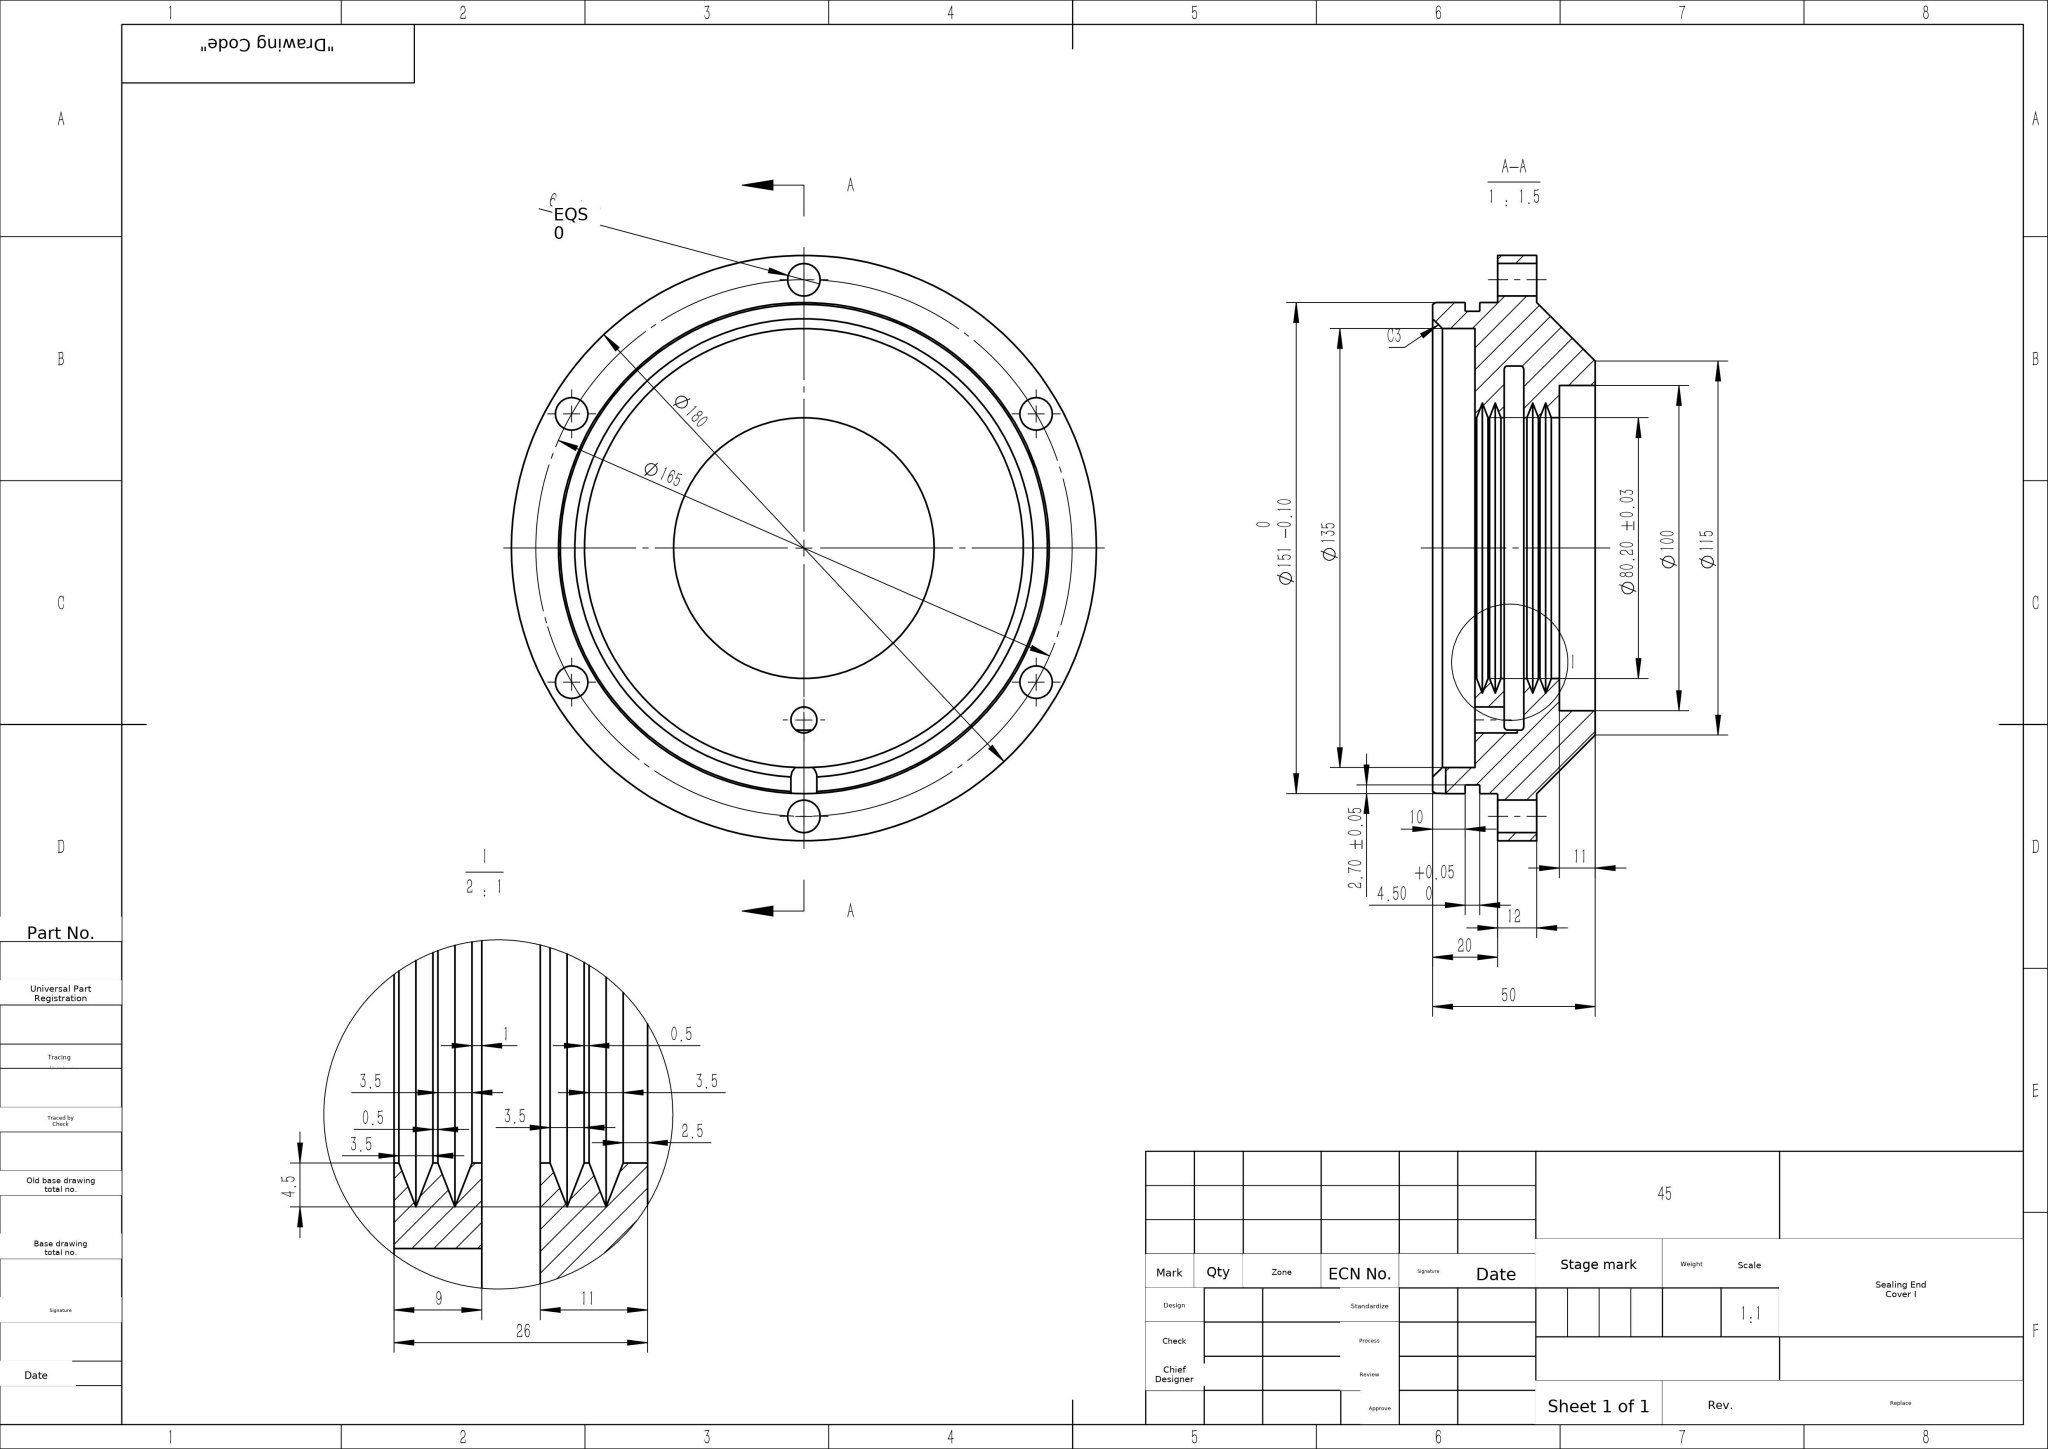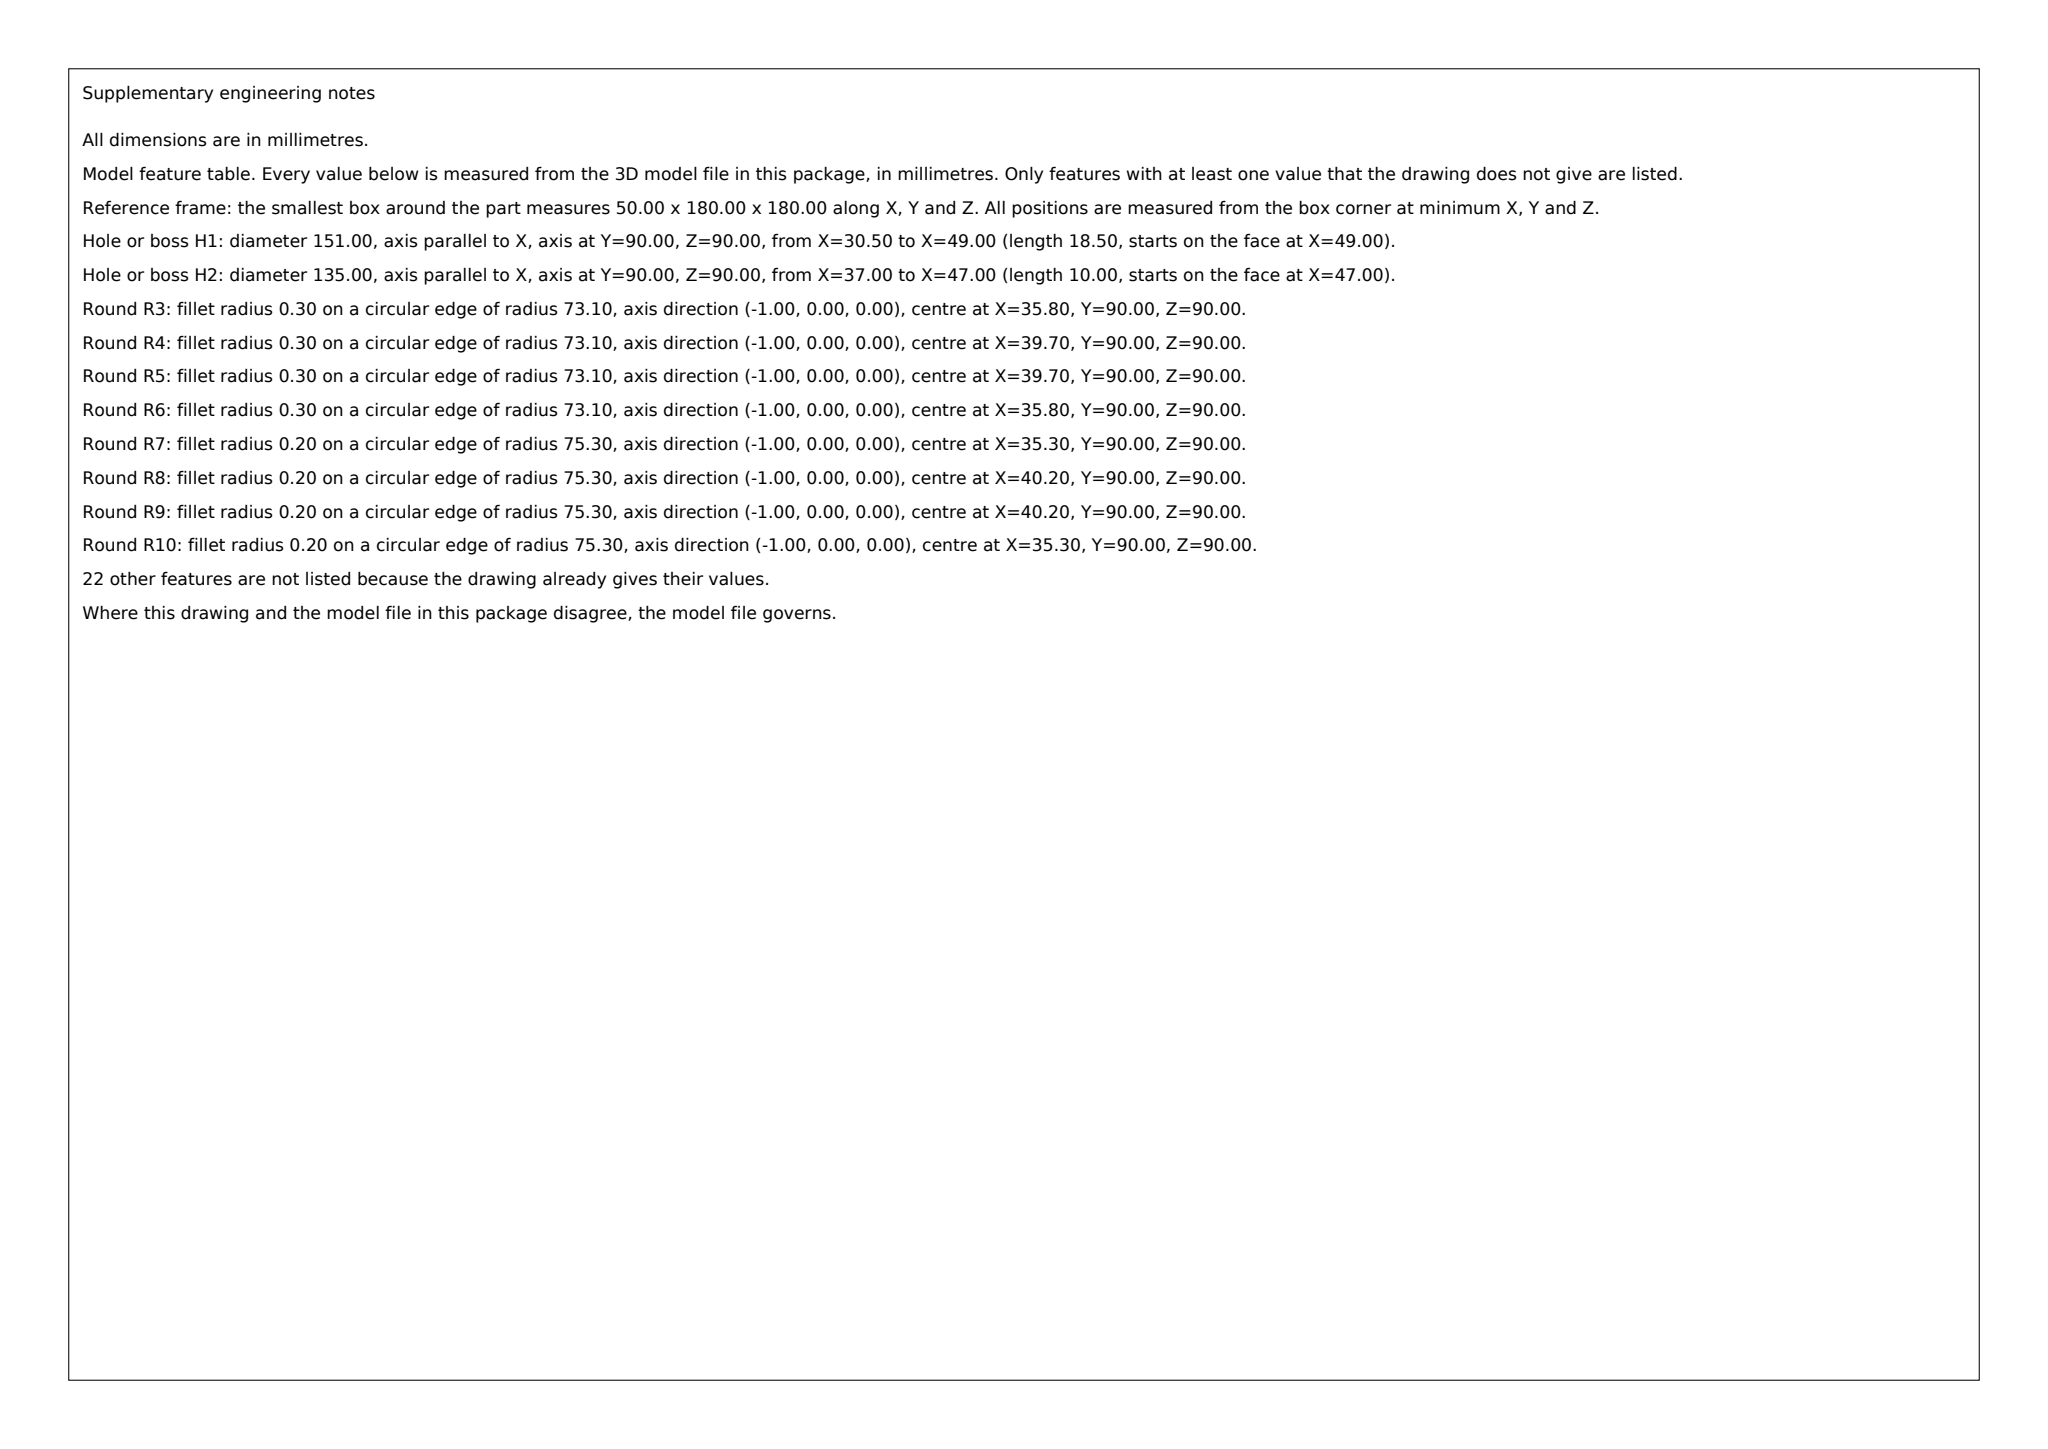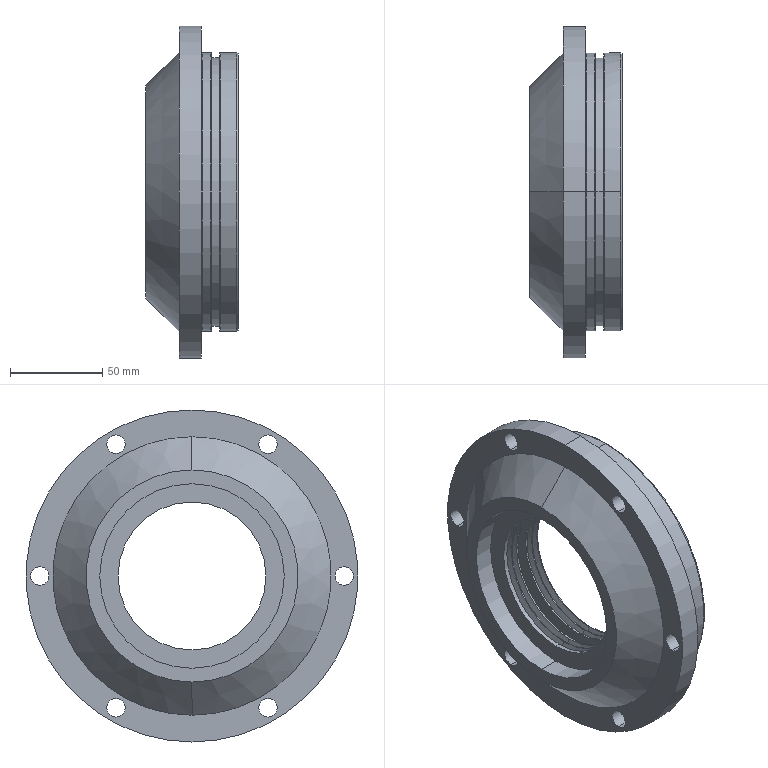Part | SolidWorks | mm | 1 solid | 91 faces | box 50 x 180 x 180 mm | volume 460431 mm3 | cylinder 41 | cone 24 | torus 15 | plane 11 | commonest cylinder face diameters 10 x12 80.2 x12 151 x4 8 x3 100 x2 180 x2 145.6 x2 112 x2
build123d program:
from build123d import *

# Parameters (mm, degrees)
SKETCH2_R          = 5
CUT_EXTRUDE1_DEPTH = 131.767
CHAMFER1_SIZE      = 3
SKETCH3_R          = 4
CUT_EXTRUDE2_DEPTH = 13
SKETCH4_R          = 4
CUT_EXTRUDE3_DEPTH = 134.12


with BuildPart() as part:
    # Sketch1 → Revolve1 (revolve)
    with BuildSketch(Plane.XY, mode=Mode.PRIVATE) as revolve1_sk:
        with BuildLine():
            Line((7, 90), (19, 90))
            Line((19, 90), (19, 76))
            ThreePointArc((19, 76), (19.146, 75.646), (19.5, 75.5))
            Line((19.5, 75.5), (24.3, 75.5))
            ThreePointArc((24.3, 75.5), (24.441, 75.441), (24.5, 75.3))
            Line((24.5, 75.3), (24.5, 73.1))
            ThreePointArc((24.5, 73.1), (24.588, 72.888), (24.8, 72.8))
            Line((24.8, 72.8), (28.7, 72.8))
            ThreePointArc((28.7, 72.8), (28.912, 72.888), (29, 73.1))
            Line((29, 73.1), (29, 75.3))
            ThreePointArc((29, 75.3), (29.059, 75.441), (29.2, 75.5))
            Line((29.2, 75.5), (38, 75.5))
            Line((38, 75.5), (39, 74.923))
            Line((39, 74.923), (39, 67.5))
            Line((39, 67.5), (26, 67.5))
            Line((26, 67.5), (26, 40.1))
            Line((26, 40.1), (25.5, 40.1))
            Line((25.5, 40.1), (23.75, 44.6))
            Line((23.75, 44.6), (22, 40.1))
            Line((22, 40.1), (21.5, 40.1))
            Line((21.5, 40.1), (19.75, 44.6))
            Line((19.75, 44.6), (18, 40.1))
            Line((18, 40.1), (17, 40.1))
            Line((17, 40.1), (17, 55))
            ThreePointArc((17, 55), (16.707, 55.707), (16, 56))
            Line((16, 56), (12, 56))
            ThreePointArc((12, 56), (11.293, 55.707), (11, 55))
            Line((11, 55), (11, 40.1))
            Line((11, 40.1), (10, 40.1))
            Line((10, 40.1), (8.25, 44.6))
            Line((8.25, 44.6), (6.5, 40.1))
            Line((6.5, 40.1), (6, 40.1))
            Line((6, 40.1), (4.25, 44.6))
            Line((4.25, 44.6), (2.5, 40.1))
            Line((2.5, 40.1), (0, 40.1))
            Line((0, 40.1), (0, 50))
            Line((0, 50), (-11, 50))
            Line((-11, 50), (-11, 57.5))
            Line((-11, 57.5), (7, 75.5))
            Line((7, 75.5), (7, 90))
        make_face()
    revolve(revolve1_sk.sketch.rotate(Axis((0, 0, 0), (1, 0, 0)), 90), axis=Axis((0, 0, 0), (1, 0, 0)))

    # Sketch2 → Cut-Extrude1 (cut, through all)
    with BuildSketch(Plane(origin=(19, 0, 0), x_dir=(0, 0, -1), z_dir=(1, 0, 0))):
        with Locations((0, 82.5)):
            Circle(SKETCH2_R)
        with Locations((71.447, 41.25)):
            Circle(SKETCH2_R)
        with Locations((71.447, -41.25)):
            Circle(SKETCH2_R)
        with Locations((0, -82.5)):
            Circle(SKETCH2_R)
        with Locations((-71.447, -41.25)):
            Circle(SKETCH2_R)
        with Locations((-71.447, 41.25)):
            Circle(SKETCH2_R)
    extrude(amount=-CUT_EXTRUDE1_DEPTH, mode=Mode.SUBTRACT)

    # Chamfer1
    chamfer1_edges = [part.edges().sort_by_distance(p)[0] for p in [
        (39, 0, -67.5),
    ]]
    chamfer(chamfer1_edges, length=CHAMFER1_SIZE)

    # Sketch3 → Cut-Extrude2 (cut)
    with BuildSketch(Plane(origin=(26, 0, 0), x_dir=(0, 0, -1), z_dir=(1, 0, 0))):
        with Locations((0, 52.866)):
            Circle(SKETCH3_R)
    extrude(amount=-CUT_EXTRUDE2_DEPTH, mode=Mode.SUBTRACT)

    # Sketch4 → Cut-Extrude3 (cut, through all)
    with BuildSketch(Plane(origin=(0, 0, 0), x_dir=(1, 0, 0), z_dir=(0, 1, 0))):
        with Locations((39, 0)):
            Circle(SKETCH4_R)
    extrude(amount=CUT_EXTRUDE3_DEPTH, mode=Mode.SUBTRACT)


solid = part.part